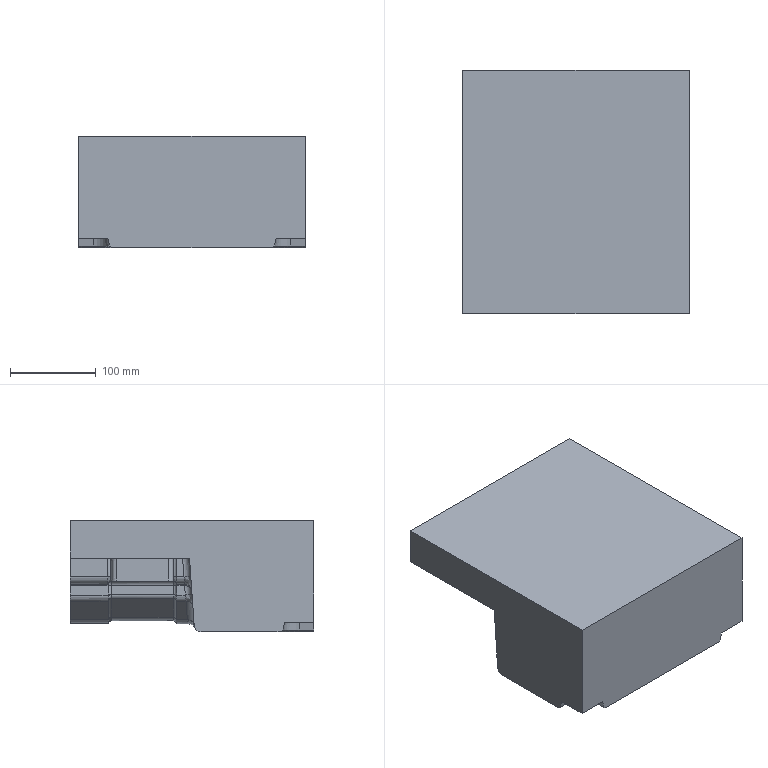CAM job | NX | mm | 3-axis | 1 set-up | 5 operations | part box 264 x 284 x 130
set-up 1
1. Cavity Milling | Mill Mill5 D50R5 | CAVITY_MILL | path 154518.782 mm | 61.482 min
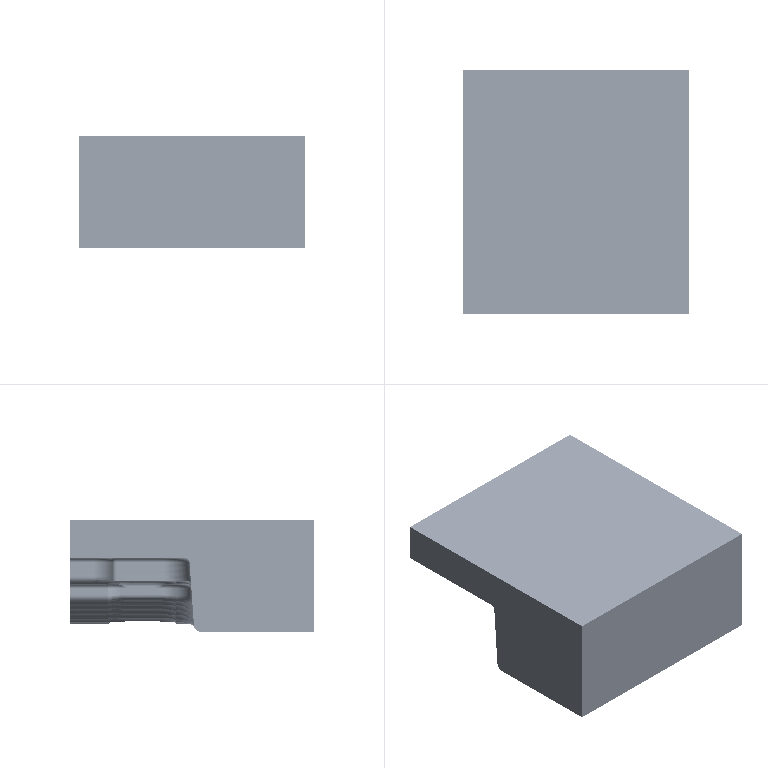2. Cavity Milling | Mill Mill5 D25R5 | FU10 | path 101115.234 mm | 40.873 min
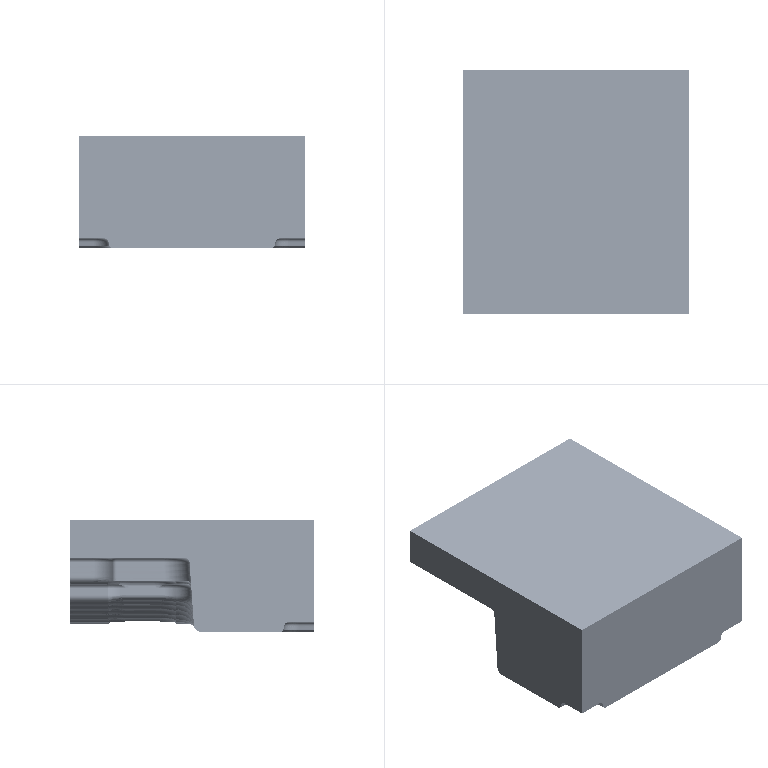3. Z-Level Milling | Mill Mill5 D10 | ZLEVEL_PROFILE | path 6371.899 mm | 2.459 min
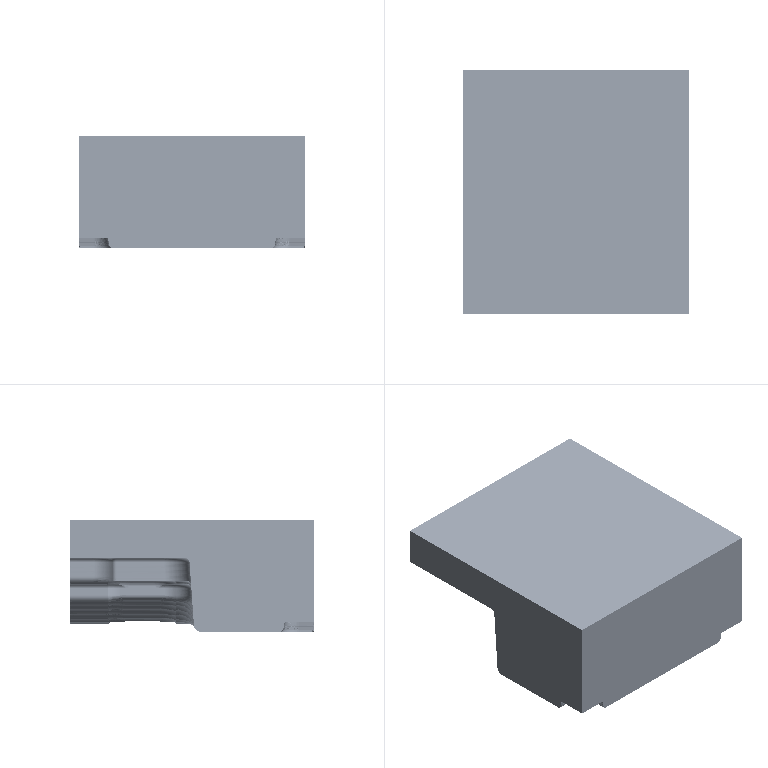4. Face Milling | Mill Mill5 D25R5 | FACE_MILLING | path 599.544 mm | 0.1628 min
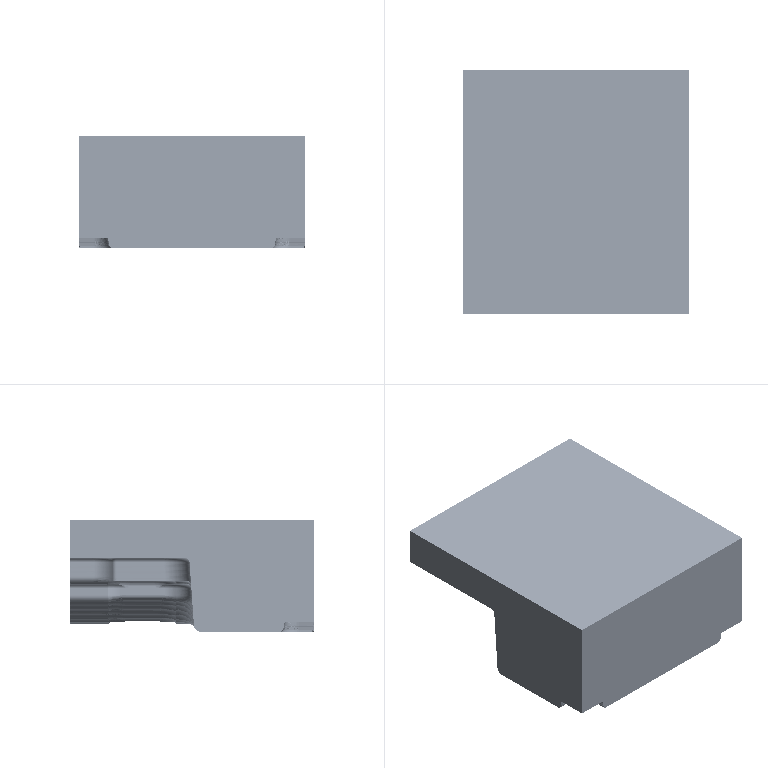5. Cavity Milling | Mill Mill5 D10 | CAVITY_MILL_1 | path 78929.957 mm | 27.407 min